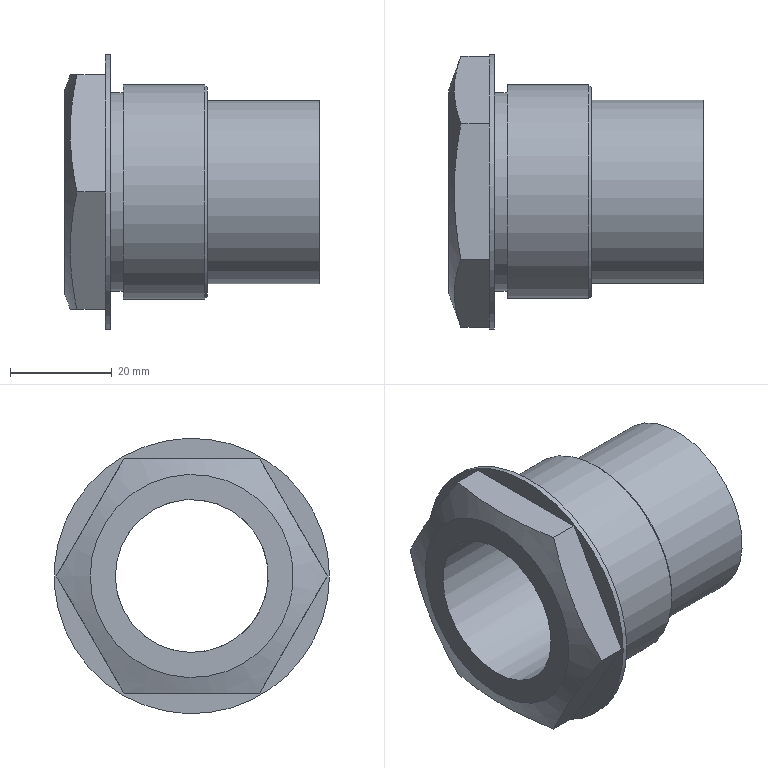Component | NX | PLUNGER_SLEEVE | 1 solid | 20 faces | volume 29320 mm3 | plane 12 | cylinder 5 | cone 3 | commonest cylinder face diameters 36 x1 42 x1 39 x1 54 x1 30 x1